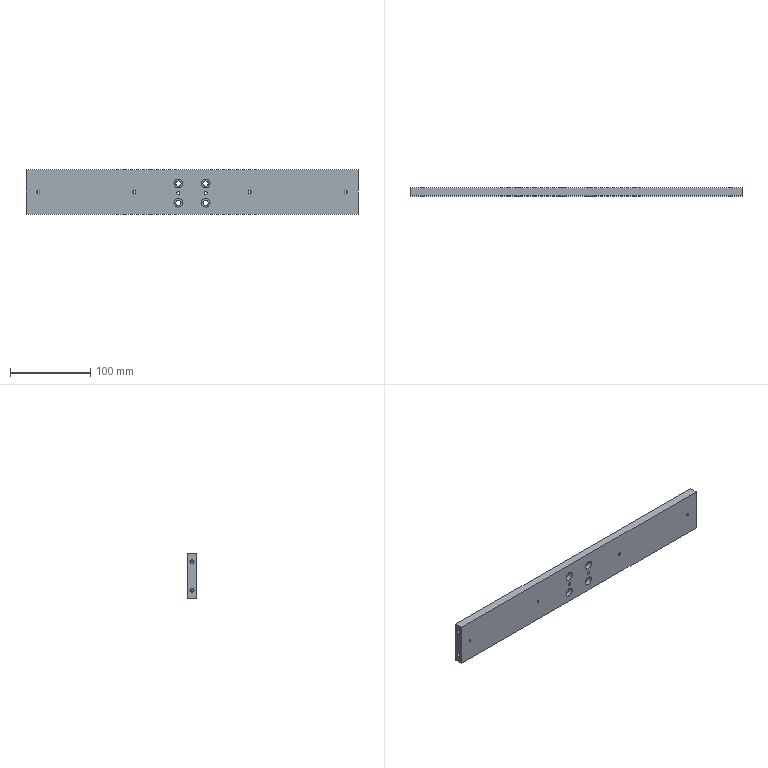Component | SolidWorks | MGPM25-20Z-A93LAssembly-1_30-31A-1 | 1 solid | 54 faces | box 414 x 10 x 55 mm | volume 222904 mm3 | cylinder 36 | plane 10 | cone 8 | commonest cylinder face diameters 6.6 x8 11 x8 5 x8 3.3 x8 4 x4
build123d program:
from build123d import *

# Parameters (mm, degrees)
EXTRUDE1_DEPTH                                       = 10
M4_TAPPED_HOLE1_D                                    = 3.3
M4_TAPPED_HOLE1_DEPTH                                = 11.5
M4_TAPPED_HOLE1_TIP                                  = 0.9914
M6_TAPPED_HOLE1_D                                    = 5
M6_TAPPED_HOLE1_DEPTH                                = 17
M6_TAPPED_HOLE1_TIP                                  = 1.502
M6_TAPPED_HOLE2_D                                    = 5
M6_TAPPED_HOLE2_DEPTH                                = 17
M6_TAPPED_HOLE2_TIP                                  = 1.502
COUNTERBORE_FOR_M6_HEXAGON_SOCKET_HEAD_C_D           = 6.6
COUNTERBORE_FOR_M6_HEXAGON_SOCKET_HEAD_C_CBORE_D     = 11
COUNTERBORE_FOR_M6_HEXAGON_SOCKET_HEAD_C_CBORE_DEPTH = 6
SKETCH17_R                                           = 2
CUT_EXTRUDE2_DEPTH                                   = 20


with BuildPart() as part:
    # Sketch1 → Extrude1 (new body)
    with BuildSketch(Plane.XY):
        Polygon((-207, 55), (207, 55), (207, 0), (-51.5, 0), (-207, 0), align=None)
    extrude(amount=EXTRUDE1_DEPTH)

    # M4 Tapped Hole1
    with Locations(Plane.XY.offset(10)):
        with Locations((-72, 27.5), (-192, 27.5), (192, 27.5), (72, 27.5)):
            Hole(M4_TAPPED_HOLE1_D / 2, depth=M4_TAPPED_HOLE1_DEPTH)
            with Locations((0, 0, -(M4_TAPPED_HOLE1_DEPTH + M4_TAPPED_HOLE1_TIP / 2))):  # 118° drill point
                Cone(0, M4_TAPPED_HOLE1_D / 2, M4_TAPPED_HOLE1_TIP, mode=Mode.SUBTRACT)

    # M6 Tapped Hole1
    with Locations(Plane(origin=(207, 0, 0), x_dir=(0, 0, -1), z_dir=(1, 0, 0))):
        with Locations((-5, 45), (-5, 10)):
            Hole(M6_TAPPED_HOLE1_D / 2, depth=M6_TAPPED_HOLE1_DEPTH)
            with Locations((0, 0, -(M6_TAPPED_HOLE1_DEPTH + M6_TAPPED_HOLE1_TIP / 2))):  # 118° drill point
                Cone(0, M6_TAPPED_HOLE1_D / 2, M6_TAPPED_HOLE1_TIP, mode=Mode.SUBTRACT)

    # M6 Tapped Hole2
    with Locations(Plane.ZY.offset(207)):
        with Locations((5, 45), (5, 10)):
            Hole(M6_TAPPED_HOLE2_D / 2, depth=M6_TAPPED_HOLE2_DEPTH)
            with Locations((0, 0, -(M6_TAPPED_HOLE2_DEPTH + M6_TAPPED_HOLE2_TIP / 2))):  # 118° drill point
                Cone(0, M6_TAPPED_HOLE2_D / 2, M6_TAPPED_HOLE2_TIP, mode=Mode.SUBTRACT)

    # Counterbore for M6 Hexagon Socket Head C (through all)
    with Locations(Plane(origin=(0, 0, 0), x_dir=(-1, 0, 0), z_dir=(0, 0, -1))):
        with Locations((-17, 38), (17, 38), (-17, 14), (17, 14)):
            CounterBoreHole(COUNTERBORE_FOR_M6_HEXAGON_SOCKET_HEAD_C_D / 2, COUNTERBORE_FOR_M6_HEXAGON_SOCKET_HEAD_C_CBORE_D / 2, COUNTERBORE_FOR_M6_HEXAGON_SOCKET_HEAD_C_CBORE_DEPTH)

    # Sketch17 → Cut-Extrude2 (cut)
    with BuildSketch(Plane.XY.offset(10)):
        with Locations((17, 26)):
            Circle(SKETCH17_R)
        with Locations((-17, 26)):
            Circle(SKETCH17_R)
    extrude(amount=-CUT_EXTRUDE2_DEPTH, mode=Mode.SUBTRACT)


solid = part.part

# Placed as in the assembly
solid = solid.moved(Location((-649.208, -12.092, 105.188), (-90, 0, 180)))